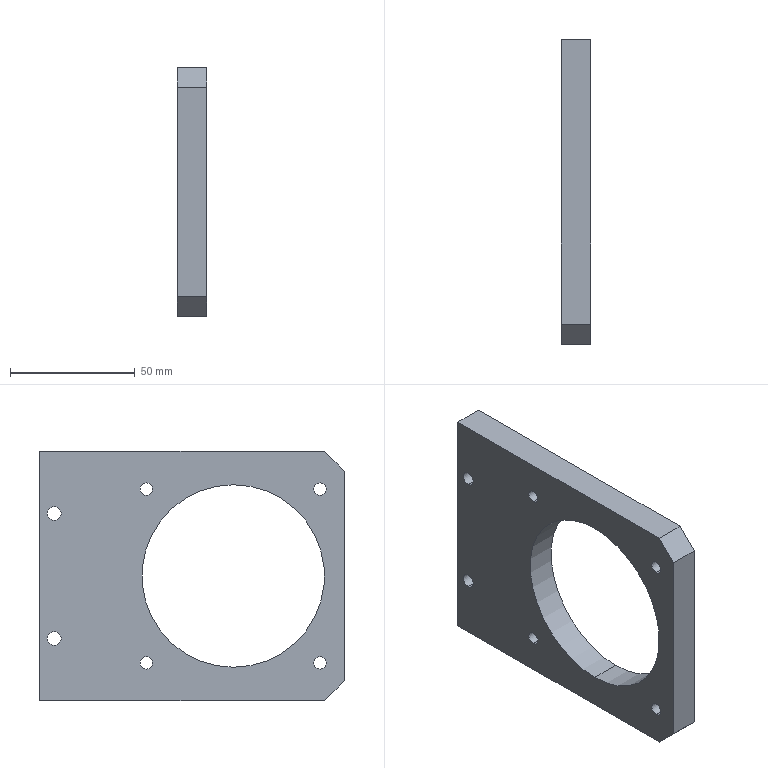Component | SolidWorks | ChainPartMotorMount-1 | 1 solid | 22 faces | box 11.8 x 122 x 99.8 mm | volume 92042 mm3 | cylinder 14 | plane 8 | commonest cylinder face diameters 5 x8 5.5 x4 73 x2
build123d program:
from build123d import *

# Parameters (mm, degrees)
SKETCH1_W           = 99.8
SKETCH1_H           = 122
BOSS_EXTRUDE1_DEPTH = 11.8
SKETCH2_R           = 36.5
CUT_EXTRUDE1_DEPTH  = 80.688
SKETCH3_R           = 1.5
CUT_EXTRUDE2_DEPTH  = 80.688
M5_TAPPED_HOLE1_D   = 5
SKETCH6_R           = 2.75
CUT_EXTRUDE3_DEPTH  = 80.688
CHAMFER1_SIZE       = 8


with BuildPart() as part:
    # Sketch1 → Boss-Extrude1 (new body)
    with BuildSketch(Plane.XY):
        Rectangle(SKETCH1_W, SKETCH1_H)
    extrude(amount=BOSS_EXTRUDE1_DEPTH)

    # Sketch2 → Cut-Extrude1 (cut, through all)
    with BuildSketch(Plane.XY.offset(11.8)):
        with Locations((0, 16.5)):
            Circle(SKETCH2_R)
    extrude(amount=-CUT_EXTRUDE1_DEPTH, mode=Mode.SUBTRACT)

    # Sketch3 → Cut-Extrude2 (cut, through all)
    with BuildSketch(Plane.XY.offset(11.8)):
        with Locations((34.75, 51.25)):
            Circle(SKETCH3_R)
        with Locations((-34.75, 51.25)):
            Circle(SKETCH3_R)
        with Locations((-34.75, -18.25)):
            Circle(SKETCH3_R)
        with Locations((34.75, -18.25)):
            Circle(SKETCH3_R)
    extrude(amount=-CUT_EXTRUDE2_DEPTH, mode=Mode.SUBTRACT)

    # M5 Tapped Hole1 (through all)
    with Locations(Plane.XY.offset(11.8)):
        with Locations((-34.75, 51.25), (34.75, 51.25), (34.75, -18.25), (-34.75, -18.25)):
            Hole(M5_TAPPED_HOLE1_D / 2)

    # Sketch6 → Cut-Extrude3 (cut, through all)
    with BuildSketch(Plane.XY.offset(11.8)):
        with Locations((-25, -55.1)):
            Circle(SKETCH6_R)
        with Locations((25, -55.1)):
            Circle(SKETCH6_R)
    extrude(amount=-CUT_EXTRUDE3_DEPTH, mode=Mode.SUBTRACT)

    # Chamfer1
    chamfer1_edges = [part.edges().sort_by_distance(p)[0] for p in [
        (-49.9, 61, 5.9),
        (49.9, 61, 5.9),
    ]]
    chamfer(chamfer1_edges, length=CHAMFER1_SIZE)


solid = part.part

# Placed as in the assembly
solid = solid.moved(Location((228.837, 13.937, -35.304), (180, 90, 0)))